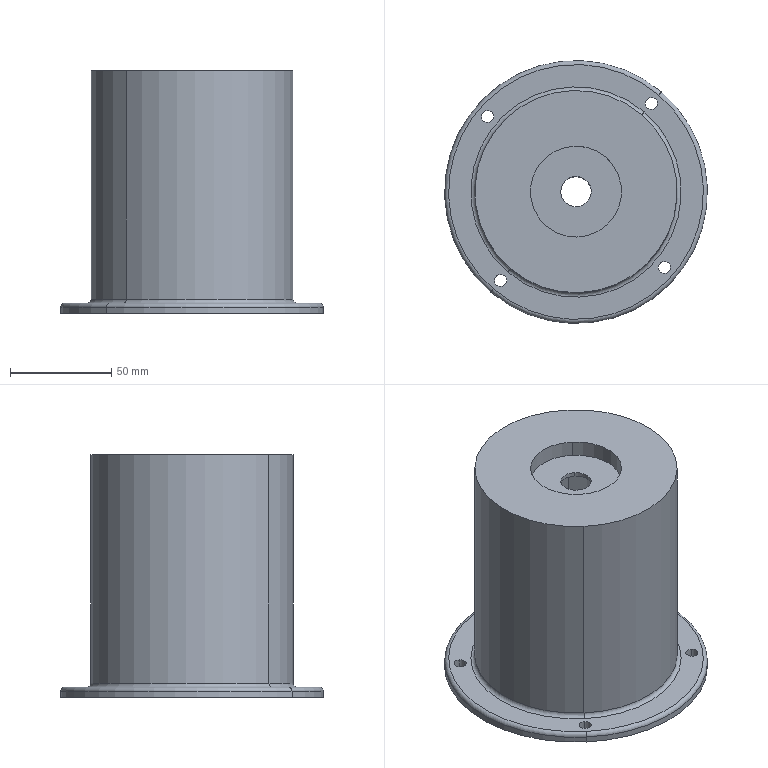Component | SolidWorks | FormingWheelMountingCover-2 | 1 solid | 41 faces | volume 213947 mm3 | cylinder 26 | plane 9 | torus 6 | commonest cylinder face diameters 6 x8 45 x4 15 x4 95 x4 130 x2 50 x2 100 x2